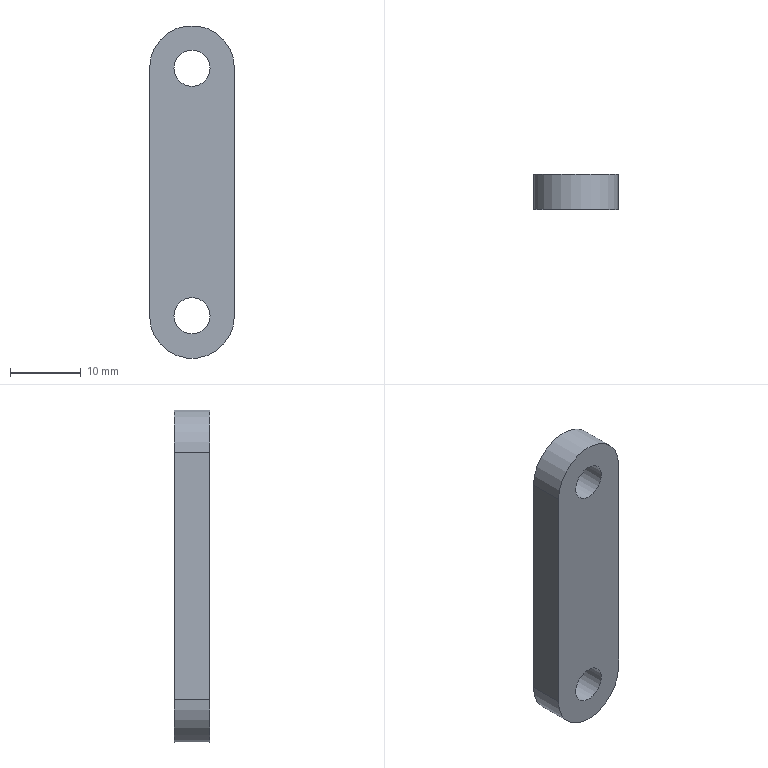Component | NX | SHORT_LINK | 1 solid | 8 faces | box 12 x 5 x 47 mm | volume 2461 mm3 | plane 4 | cylinder 4 | commonest cylinder face diameters 12 x2 5.1 x2
STEP:
#1=CARTESIAN_POINT('',(0.,0.,0.));
#2=DIRECTION('',(0.,0.,1.));
#3=DIRECTION('',(1.,0.,0.));
#4=AXIS2_PLACEMENT_3D('',#1,#2,#3);
#5=CARTESIAN_POINT('',(-34.,3.5,67.45));
#6=VERTEX_POINT('',#5);
#7=CARTESIAN_POINT('',(-34.,3.5,102.45));
#8=VERTEX_POINT('',#7);
#9=CARTESIAN_POINT('',(-34.,3.5,67.45));
#10=DIRECTION('',(-0.,0.,1.));
#11=VECTOR('',#10,1.);
#12=LINE('',#9,#11);
#13=CARTESIAN_POINT('',(-34.,-1.5,67.45));
#14=DIRECTION('',(-1.,0.,-0.));
#15=DIRECTION('',(0.,0.,-1.));
#16=AXIS2_PLACEMENT_3D('',#13,#14,#15);
#17=PLANE('',#16);
#18=CARTESIAN_POINT('',(0.,-5.));
#19=DIRECTION('',(-1.,0.));
#20=VECTOR('',#19,1.);
#21=LINE('',#18,#20);
#22=(GEOMETRIC_REPRESENTATION_CONTEXT(2)PARAMETRIC_REPRESENTATION_CONTEXT()REPRESENTATION_CONTEXT('',''));
#23=DEFINITIONAL_REPRESENTATION('',(#21),#22);
#24=PCURVE('',#17,#23);
#25=CARTESIAN_POINT('',(-40.,3.5,102.45));
#26=DIRECTION('',(0.,-1.,0.));
#27=DIRECTION('',(1.,0.,0.));
#28=AXIS2_PLACEMENT_3D('',#25,#26,#27);
#29=PLANE('',#28);
#30=CARTESIAN_POINT('',(6.,-35.));
#31=DIRECTION('',(-0.,1.));
#32=VECTOR('',#31,1.);
#33=LINE('',#30,#32);
#34=(GEOMETRIC_REPRESENTATION_CONTEXT(2)PARAMETRIC_REPRESENTATION_CONTEXT()REPRESENTATION_CONTEXT('',''));
#35=DEFINITIONAL_REPRESENTATION('',(#33),#34);
#36=PCURVE('',#29,#35);
#37=SURFACE_CURVE('',#12,(#24,#36),.PCURVE_S1.);
#38=EDGE_CURVE('',#6,#8,#37,.T.);
#39=ORIENTED_EDGE('',*,*,#38,.T.);
#40=CARTESIAN_POINT('',(-34.,-1.5,102.45));
#41=VERTEX_POINT('',#40);
#42=CARTESIAN_POINT('',(-34.,-1.5,102.45));
#43=DIRECTION('',(0.,1.,0.));
#44=VECTOR('',#43,1.);
#45=LINE('',#42,#44);
#46=CARTESIAN_POINT('',(-35.,0.));
#47=DIRECTION('',(0.,-1.));
#48=VECTOR('',#47,1.);
#49=LINE('',#46,#48);
#50=(GEOMETRIC_REPRESENTATION_CONTEXT(2)PARAMETRIC_REPRESENTATION_CONTEXT()REPRESENTATION_CONTEXT('',''));
#51=DEFINITIONAL_REPRESENTATION('',(#49),#50);
#52=PCURVE('',#17,#51);
#53=CARTESIAN_POINT('',(-40.,-1.5,102.45));
#54=DIRECTION('',(0.,1.,0.));
#55=DIRECTION('',(-1.,0.,0.));
#56=AXIS2_PLACEMENT_3D('',#53,#54,#55);
#57=CYLINDRICAL_SURFACE('',#56,6.);
#58=CARTESIAN_POINT('',(3.142,0.));
#59=DIRECTION('',(0.,1.));
#60=VECTOR('',#59,1.);
#61=LINE('',#58,#60);
#62=(GEOMETRIC_REPRESENTATION_CONTEXT(2)PARAMETRIC_REPRESENTATION_CONTEXT()REPRESENTATION_CONTEXT('',''));
#63=DEFINITIONAL_REPRESENTATION('',(#61),#62);
#64=PCURVE('',#57,#63);
#65=SURFACE_CURVE('',#45,(#52,#64),.PCURVE_S1.);
#66=EDGE_CURVE('',#41,#8,#65,.T.);
#67=ORIENTED_EDGE('',*,*,#66,.F.);
#68=CARTESIAN_POINT('',(-34.,-1.5,67.45));
#69=VERTEX_POINT('',#68);
#70=CARTESIAN_POINT('',(-34.,-1.5,67.45));
#71=DIRECTION('',(-0.,0.,1.));
#72=VECTOR('',#71,1.);
#73=LINE('',#70,#72);
#74=CARTESIAN_POINT('',(0.,0.));
#75=DIRECTION('',(-1.,0.));
#76=VECTOR('',#75,1.);
#77=LINE('',#74,#76);
#78=(GEOMETRIC_REPRESENTATION_CONTEXT(2)PARAMETRIC_REPRESENTATION_CONTEXT()REPRESENTATION_CONTEXT('',''));
#79=DEFINITIONAL_REPRESENTATION('',(#77),#78);
#80=PCURVE('',#17,#79);
#81=CARTESIAN_POINT('',(-40.,-1.5,102.45));
#82=DIRECTION('',(0.,-1.,0.));
#83=DIRECTION('',(1.,0.,0.));
#84=AXIS2_PLACEMENT_3D('',#81,#82,#83);
#85=PLANE('',#84);
#86=CARTESIAN_POINT('',(6.,-35.));
#87=DIRECTION('',(-0.,1.));
#88=VECTOR('',#87,1.);
#89=LINE('',#86,#88);
#90=(GEOMETRIC_REPRESENTATION_CONTEXT(2)PARAMETRIC_REPRESENTATION_CONTEXT()REPRESENTATION_CONTEXT('',''));
#91=DEFINITIONAL_REPRESENTATION('',(#89),#90);
#92=PCURVE('',#85,#91);
#93=SURFACE_CURVE('',#73,(#80,#92),.PCURVE_S1.);
#94=EDGE_CURVE('',#69,#41,#93,.T.);
#95=ORIENTED_EDGE('',*,*,#94,.F.);
#96=CARTESIAN_POINT('',(-34.,-1.5,67.45));
#97=DIRECTION('',(0.,1.,0.));
#98=VECTOR('',#97,1.);
#99=LINE('',#96,#98);
#100=CARTESIAN_POINT('',(0.,0.));
#101=DIRECTION('',(0.,-1.));
#102=VECTOR('',#101,1.);
#103=LINE('',#100,#102);
#104=(GEOMETRIC_REPRESENTATION_CONTEXT(2)PARAMETRIC_REPRESENTATION_CONTEXT()REPRESENTATION_CONTEXT('',''));
#105=DEFINITIONAL_REPRESENTATION('',(#103),#104);
#106=PCURVE('',#17,#105);
#107=CARTESIAN_POINT('',(-40.,-1.5,67.45));
#108=DIRECTION('',(0.,1.,0.));
#109=DIRECTION('',(-1.,0.,0.));
#110=AXIS2_PLACEMENT_3D('',#107,#108,#109);
#111=CYLINDRICAL_SURFACE('',#110,6.);
#112=CARTESIAN_POINT('',(3.142,0.));
#113=DIRECTION('',(0.,1.));
#114=VECTOR('',#113,1.);
#115=LINE('',#112,#114);
#116=(GEOMETRIC_REPRESENTATION_CONTEXT(2)PARAMETRIC_REPRESENTATION_CONTEXT()REPRESENTATION_CONTEXT('',''));
#117=DEFINITIONAL_REPRESENTATION('',(#115),#116);
#118=PCURVE('',#111,#117);
#119=SURFACE_CURVE('',#99,(#106,#118),.PCURVE_S1.);
#120=EDGE_CURVE('',#69,#6,#119,.T.);
#121=ORIENTED_EDGE('',*,*,#120,.T.);
#122=EDGE_LOOP('',(#39,#67,#95,#121));
#123=FACE_BOUND('',#122,.T.);
#124=ADVANCED_FACE('',(#123),#17,.F.);
#125=CARTESIAN_POINT('',(-46.,3.5,102.45));
#126=VERTEX_POINT('',#125);
#127=CARTESIAN_POINT('',(-40.,3.5,102.45));
#128=DIRECTION('',(0.,-1.,0.));
#129=DIRECTION('',(1.,0.,0.));
#130=AXIS2_PLACEMENT_3D('',#127,#128,#129);
#131=CIRCLE('',#130,6.);
#132=CARTESIAN_POINT('',(3.142,5.));
#133=DIRECTION('',(-1.,0.));
#134=VECTOR('',#133,1.);
#135=LINE('',#132,#134);
#136=(GEOMETRIC_REPRESENTATION_CONTEXT(2)PARAMETRIC_REPRESENTATION_CONTEXT()REPRESENTATION_CONTEXT('',''));
#137=DEFINITIONAL_REPRESENTATION('',(#135),#136);
#138=PCURVE('',#57,#137);
#139=CARTESIAN_POINT('',(0.,0.));
#140=DIRECTION('',(1.,0.));
#141=AXIS2_PLACEMENT_2D('',#139,#140);
#142=CIRCLE('',#141,6.);
#143=(GEOMETRIC_REPRESENTATION_CONTEXT(2)PARAMETRIC_REPRESENTATION_CONTEXT()REPRESENTATION_CONTEXT('',''));
#144=DEFINITIONAL_REPRESENTATION('',(#142),#143);
#145=PCURVE('',#29,#144);
#146=SURFACE_CURVE('',#131,(#138,#145),.PCURVE_S1.);
#147=EDGE_CURVE('',#8,#126,#146,.T.);
#148=ORIENTED_EDGE('',*,*,#147,.T.);
#149=CARTESIAN_POINT('',(-46.,-1.5,102.45));
#150=VERTEX_POINT('',#149);
#151=CARTESIAN_POINT('',(-46.,-1.5,102.45));
#152=DIRECTION('',(0.,1.,0.));
#153=VECTOR('',#152,1.);
#154=LINE('',#151,#153);
#155=CARTESIAN_POINT('',(0.,0.));
#156=DIRECTION('',(0.,1.));
#157=VECTOR('',#156,1.);
#158=LINE('',#155,#157);
#159=(GEOMETRIC_REPRESENTATION_CONTEXT(2)PARAMETRIC_REPRESENTATION_CONTEXT()REPRESENTATION_CONTEXT('',''));
#160=DEFINITIONAL_REPRESENTATION('',(#158),#159);
#161=PCURVE('',#57,#160);
#162=CARTESIAN_POINT('',(-46.,-1.5,102.45));
#163=DIRECTION('',(1.,0.,0.));
#164=DIRECTION('',(-0.,0.,1.));
#165=AXIS2_PLACEMENT_3D('',#162,#163,#164);
#166=PLANE('',#165);
#167=CARTESIAN_POINT('',(0.,0.));
#168=DIRECTION('',(0.,-1.));
#169=VECTOR('',#168,1.);
#170=LINE('',#167,#169);
#171=(GEOMETRIC_REPRESENTATION_CONTEXT(2)PARAMETRIC_REPRESENTATION_CONTEXT()REPRESENTATION_CONTEXT('',''));
#172=DEFINITIONAL_REPRESENTATION('',(#170),#171);
#173=PCURVE('',#166,#172);
#174=SURFACE_CURVE('',#154,(#161,#173),.PCURVE_S1.);
#175=EDGE_CURVE('',#150,#126,#174,.T.);
#176=ORIENTED_EDGE('',*,*,#175,.F.);
#177=CARTESIAN_POINT('',(-40.,-1.5,102.45));
#178=DIRECTION('',(0.,-1.,0.));
#179=DIRECTION('',(1.,0.,0.));
#180=AXIS2_PLACEMENT_3D('',#177,#178,#179);
#181=CIRCLE('',#180,6.);
#182=CARTESIAN_POINT('',(3.142,0.));
#183=DIRECTION('',(-1.,0.));
#184=VECTOR('',#183,1.);
#185=LINE('',#182,#184);
#186=(GEOMETRIC_REPRESENTATION_CONTEXT(2)PARAMETRIC_REPRESENTATION_CONTEXT()REPRESENTATION_CONTEXT('',''));
#187=DEFINITIONAL_REPRESENTATION('',(#185),#186);
#188=PCURVE('',#57,#187);
#189=CARTESIAN_POINT('',(0.,0.));
#190=DIRECTION('',(1.,0.));
#191=AXIS2_PLACEMENT_2D('',#189,#190);
#192=CIRCLE('',#191,6.);
#193=(GEOMETRIC_REPRESENTATION_CONTEXT(2)PARAMETRIC_REPRESENTATION_CONTEXT()REPRESENTATION_CONTEXT('',''));
#194=DEFINITIONAL_REPRESENTATION('',(#192),#193);
#195=PCURVE('',#85,#194);
#196=SURFACE_CURVE('',#181,(#188,#195),.PCURVE_S1.);
#197=EDGE_CURVE('',#41,#150,#196,.T.);
#198=ORIENTED_EDGE('',*,*,#197,.F.);
#199=ORIENTED_EDGE('',*,*,#66,.T.);
#200=EDGE_LOOP('',(#148,#176,#198,#199));
#201=FACE_BOUND('',#200,.T.);
#202=ADVANCED_FACE('',(#201),#57,.T.);
#203=CARTESIAN_POINT('',(-46.,3.5,67.45));
#204=VERTEX_POINT('',#203);
#205=CARTESIAN_POINT('',(-46.,3.5,102.45));
#206=DIRECTION('',(0.,0.,-1.));
#207=VECTOR('',#206,1.);
#208=LINE('',#205,#207);
#209=CARTESIAN_POINT('',(0.,-5.));
#210=DIRECTION('',(-1.,0.));
#211=VECTOR('',#210,1.);
#212=LINE('',#209,#211);
#213=(GEOMETRIC_REPRESENTATION_CONTEXT(2)PARAMETRIC_REPRESENTATION_CONTEXT()REPRESENTATION_CONTEXT('',''));
#214=DEFINITIONAL_REPRESENTATION('',(#212),#213);
#215=PCURVE('',#166,#214);
#216=CARTESIAN_POINT('',(-6.,0.));
#217=DIRECTION('',(0.,-1.));
#218=VECTOR('',#217,1.);
#219=LINE('',#216,#218);
#220=(GEOMETRIC_REPRESENTATION_CONTEXT(2)PARAMETRIC_REPRESENTATION_CONTEXT()REPRESENTATION_CONTEXT('',''));
#221=DEFINITIONAL_REPRESENTATION('',(#219),#220);
#222=PCURVE('',#29,#221);
#223=SURFACE_CURVE('',#208,(#215,#222),.PCURVE_S1.);
#224=EDGE_CURVE('',#126,#204,#223,.T.);
#225=ORIENTED_EDGE('',*,*,#224,.T.);
#226=CARTESIAN_POINT('',(-46.,-1.5,67.45));
#227=VERTEX_POINT('',#226);
#228=CARTESIAN_POINT('',(-46.,-1.5,67.45));
#229=DIRECTION('',(0.,1.,0.));
#230=VECTOR('',#229,1.);
#231=LINE('',#228,#230);
#232=CARTESIAN_POINT('',(-35.,0.));
#233=DIRECTION('',(0.,-1.));
#234=VECTOR('',#233,1.);
#235=LINE('',#232,#234);
#236=(GEOMETRIC_REPRESENTATION_CONTEXT(2)PARAMETRIC_REPRESENTATION_CONTEXT()REPRESENTATION_CONTEXT('',''));
#237=DEFINITIONAL_REPRESENTATION('',(#235),#236);
#238=PCURVE('',#166,#237);
#239=CARTESIAN_POINT('',(6.283,0.));
#240=DIRECTION('',(0.,1.));
#241=VECTOR('',#240,1.);
#242=LINE('',#239,#241);
#243=(GEOMETRIC_REPRESENTATION_CONTEXT(2)PARAMETRIC_REPRESENTATION_CONTEXT()REPRESENTATION_CONTEXT('',''));
#244=DEFINITIONAL_REPRESENTATION('',(#242),#243);
#245=PCURVE('',#111,#244);
#246=SURFACE_CURVE('',#231,(#238,#245),.PCURVE_S1.);
#247=EDGE_CURVE('',#227,#204,#246,.T.);
#248=ORIENTED_EDGE('',*,*,#247,.F.);
#249=CARTESIAN_POINT('',(-46.,-1.5,102.45));
#250=DIRECTION('',(0.,0.,-1.));
#251=VECTOR('',#250,1.);
#252=LINE('',#249,#251);
#253=CARTESIAN_POINT('',(0.,0.));
#254=DIRECTION('',(-1.,0.));
#255=VECTOR('',#254,1.);
#256=LINE('',#253,#255);
#257=(GEOMETRIC_REPRESENTATION_CONTEXT(2)PARAMETRIC_REPRESENTATION_CONTEXT()REPRESENTATION_CONTEXT('',''));
#258=DEFINITIONAL_REPRESENTATION('',(#256),#257);
#259=PCURVE('',#166,#258);
#260=CARTESIAN_POINT('',(-6.,0.));
#261=DIRECTION('',(0.,-1.));
#262=VECTOR('',#261,1.);
#263=LINE('',#260,#262);
#264=(GEOMETRIC_REPRESENTATION_CONTEXT(2)PARAMETRIC_REPRESENTATION_CONTEXT()REPRESENTATION_CONTEXT('',''));
#265=DEFINITIONAL_REPRESENTATION('',(#263),#264);
#266=PCURVE('',#85,#265);
#267=SURFACE_CURVE('',#252,(#259,#266),.PCURVE_S1.);
#268=EDGE_CURVE('',#150,#227,#267,.T.);
#269=ORIENTED_EDGE('',*,*,#268,.F.);
#270=ORIENTED_EDGE('',*,*,#175,.T.);
#271=EDGE_LOOP('',(#225,#248,#269,#270));
#272=FACE_BOUND('',#271,.T.);
#273=ADVANCED_FACE('',(#272),#166,.F.);
#274=CARTESIAN_POINT('',(-37.45,-1.5,102.45));
#275=VERTEX_POINT('',#274);
#276=CARTESIAN_POINT('',(-40.,-1.5,102.45));
#277=DIRECTION('',(0.,1.,0.));
#278=DIRECTION('',(1.,0.,0.));
#279=AXIS2_PLACEMENT_3D('',#276,#277,#278);
#280=CIRCLE('',#279,2.55);
#281=CARTESIAN_POINT('',(-40.,-1.5,102.45));
#282=DIRECTION('',(0.,1.,0.));
#283=DIRECTION('',(-1.,0.,0.));
#284=AXIS2_PLACEMENT_3D('',#281,#282,#283);
#285=CYLINDRICAL_SURFACE('',#284,2.55);
#286=CARTESIAN_POINT('',(3.142,0.));
#287=DIRECTION('',(1.,0.));
#288=VECTOR('',#287,1.);
#289=LINE('',#286,#288);
#290=(GEOMETRIC_REPRESENTATION_CONTEXT(2)PARAMETRIC_REPRESENTATION_CONTEXT()REPRESENTATION_CONTEXT('',''));
#291=DEFINITIONAL_REPRESENTATION('',(#289),#290);
#292=PCURVE('',#285,#291);
#293=CARTESIAN_POINT('',(2.55,0.));
#294=CARTESIAN_POINT('',(2.55,-4.417));
#295=CARTESIAN_POINT('',(-1.275,-2.208));
#296=CARTESIAN_POINT('',(-5.1,-0.));
#297=CARTESIAN_POINT('',(-1.275,2.208));
#298=CARTESIAN_POINT('',(2.55,4.417));
#299=CARTESIAN_POINT('',(2.55,0.));
#300=(BOUNDED_CURVE()B_SPLINE_CURVE(2,(#293,#294,#295,#296,#297,#298,#299),.UNSPECIFIED.,.T.,.F.)B_SPLINE_CURVE_WITH_KNOTS((1,2,2,2,2,1),(-2.094,0.,2.094,4.189,6.283,8.378),.UNSPECIFIED.)CURVE()GEOMETRIC_REPRESENTATION_ITEM()RATIONAL_B_SPLINE_CURVE((1.,0.5,1.,0.5,1.,0.5,1.))REPRESENTATION_ITEM(''));
#301=(GEOMETRIC_REPRESENTATION_CONTEXT(2)PARAMETRIC_REPRESENTATION_CONTEXT()REPRESENTATION_CONTEXT('',''));
#302=DEFINITIONAL_REPRESENTATION('',(#300),#301);
#303=PCURVE('',#85,#302);
#304=SURFACE_CURVE('',#280,(#292,#303),.PCURVE_S1.);
#305=EDGE_CURVE('',#275,#275,#304,.T.);
#306=ORIENTED_EDGE('',*,*,#305,.T.);
#307=CARTESIAN_POINT('',(-37.45,3.5,102.45));
#308=VERTEX_POINT('',#307);
#309=CARTESIAN_POINT('',(-37.45,-1.5,102.45));
#310=CARTESIAN_POINT('',(-37.45,3.5,102.45));
#311=B_SPLINE_CURVE_WITH_KNOTS('',1,(#309,#310),.UNSPECIFIED.,.F.,.F.,(2,2),(0.,5.),.PIECEWISE_BEZIER_KNOTS.);
#312=CARTESIAN_POINT('',(9.425,0.));
#313=DIRECTION('',(0.,1.));
#314=VECTOR('',#313,1.);
#315=LINE('',#312,#314);
#316=(GEOMETRIC_REPRESENTATION_CONTEXT(2)PARAMETRIC_REPRESENTATION_CONTEXT()REPRESENTATION_CONTEXT('',''));
#317=DEFINITIONAL_REPRESENTATION('',(#315),#316);
#318=PCURVE('',#285,#317);
#319=CARTESIAN_POINT('',(3.142,0.));
#320=DIRECTION('',(0.,1.));
#321=VECTOR('',#320,1.);
#322=LINE('',#319,#321);
#323=(GEOMETRIC_REPRESENTATION_CONTEXT(2)PARAMETRIC_REPRESENTATION_CONTEXT()REPRESENTATION_CONTEXT('',''));
#324=DEFINITIONAL_REPRESENTATION('',(#322),#323);
#325=PCURVE('',#285,#324);
#326=SEAM_CURVE('',#311,(#318,#325),.PCURVE_S1.);
#327=EDGE_CURVE('',#275,#308,#326,.T.);
#328=ORIENTED_EDGE('',*,*,#327,.T.);
#329=CARTESIAN_POINT('',(-40.,3.5,102.45));
#330=DIRECTION('',(0.,1.,0.));
#331=DIRECTION('',(1.,0.,0.));
#332=AXIS2_PLACEMENT_3D('',#329,#330,#331);
#333=CIRCLE('',#332,2.55);
#334=CARTESIAN_POINT('',(3.142,5.));
#335=DIRECTION('',(1.,0.));
#336=VECTOR('',#335,1.);
#337=LINE('',#334,#336);
#338=(GEOMETRIC_REPRESENTATION_CONTEXT(2)PARAMETRIC_REPRESENTATION_CONTEXT()REPRESENTATION_CONTEXT('',''));
#339=DEFINITIONAL_REPRESENTATION('',(#337),#338);
#340=PCURVE('',#285,#339);
#341=CARTESIAN_POINT('',(2.55,0.));
#342=CARTESIAN_POINT('',(2.55,-4.417));
#343=CARTESIAN_POINT('',(-1.275,-2.208));
#344=CARTESIAN_POINT('',(-5.1,-0.));
#345=CARTESIAN_POINT('',(-1.275,2.208));
#346=CARTESIAN_POINT('',(2.55,4.417));
#347=CARTESIAN_POINT('',(2.55,0.));
#348=(BOUNDED_CURVE()B_SPLINE_CURVE(2,(#341,#342,#343,#344,#345,#346,#347),.UNSPECIFIED.,.T.,.F.)B_SPLINE_CURVE_WITH_KNOTS((1,2,2,2,2,1),(-2.094,0.,2.094,4.189,6.283,8.378),.UNSPECIFIED.)CURVE()GEOMETRIC_REPRESENTATION_ITEM()RATIONAL_B_SPLINE_CURVE((1.,0.5,1.,0.5,1.,0.5,1.))REPRESENTATION_ITEM(''));
#349=(GEOMETRIC_REPRESENTATION_CONTEXT(2)PARAMETRIC_REPRESENTATION_CONTEXT()REPRESENTATION_CONTEXT('',''));
#350=DEFINITIONAL_REPRESENTATION('',(#348),#349);
#351=PCURVE('',#29,#350);
#352=SURFACE_CURVE('',#333,(#340,#351),.PCURVE_S1.);
#353=EDGE_CURVE('',#308,#308,#352,.T.);
#354=ORIENTED_EDGE('',*,*,#353,.F.);
#355=ORIENTED_EDGE('',*,*,#327,.F.);
#356=EDGE_LOOP('',(#306,#328,#354,#355));
#357=FACE_BOUND('',#356,.F.);
#358=ADVANCED_FACE('',(#357),#285,.F.);
#359=CARTESIAN_POINT('',(-40.,3.5,67.45));
#360=DIRECTION('',(0.,-1.,0.));
#361=DIRECTION('',(1.,0.,0.));
#362=AXIS2_PLACEMENT_3D('',#359,#360,#361);
#363=CIRCLE('',#362,6.);
#364=CARTESIAN_POINT('',(9.425,5.));
#365=DIRECTION('',(-1.,0.));
#366=VECTOR('',#365,1.);
#367=LINE('',#364,#366);
#368=(GEOMETRIC_REPRESENTATION_CONTEXT(2)PARAMETRIC_REPRESENTATION_CONTEXT()REPRESENTATION_CONTEXT('',''));
#369=DEFINITIONAL_REPRESENTATION('',(#367),#368);
#370=PCURVE('',#111,#369);
#371=CARTESIAN_POINT('',(0.,-35.));
#372=DIRECTION('',(1.,0.));
#373=AXIS2_PLACEMENT_2D('',#371,#372);
#374=CIRCLE('',#373,6.);
#375=(GEOMETRIC_REPRESENTATION_CONTEXT(2)PARAMETRIC_REPRESENTATION_CONTEXT()REPRESENTATION_CONTEXT('',''));
#376=DEFINITIONAL_REPRESENTATION('',(#374),#375);
#377=PCURVE('',#29,#376);
#378=SURFACE_CURVE('',#363,(#370,#377),.PCURVE_S1.);
#379=EDGE_CURVE('',#204,#6,#378,.T.);
#380=ORIENTED_EDGE('',*,*,#379,.T.);
#381=ORIENTED_EDGE('',*,*,#120,.F.);
#382=CARTESIAN_POINT('',(-40.,-1.5,67.45));
#383=DIRECTION('',(0.,-1.,0.));
#384=DIRECTION('',(1.,0.,0.));
#385=AXIS2_PLACEMENT_3D('',#382,#383,#384);
#386=CIRCLE('',#385,6.);
#387=CARTESIAN_POINT('',(9.425,0.));
#388=DIRECTION('',(-1.,0.));
#389=VECTOR('',#388,1.);
#390=LINE('',#387,#389);
#391=(GEOMETRIC_REPRESENTATION_CONTEXT(2)PARAMETRIC_REPRESENTATION_CONTEXT()REPRESENTATION_CONTEXT('',''));
#392=DEFINITIONAL_REPRESENTATION('',(#390),#391);
#393=PCURVE('',#111,#392);
#394=CARTESIAN_POINT('',(0.,-35.));
#395=DIRECTION('',(1.,0.));
#396=AXIS2_PLACEMENT_2D('',#394,#395);
#397=CIRCLE('',#396,6.);
#398=(GEOMETRIC_REPRESENTATION_CONTEXT(2)PARAMETRIC_REPRESENTATION_CONTEXT()REPRESENTATION_CONTEXT('',''));
#399=DEFINITIONAL_REPRESENTATION('',(#397),#398);
#400=PCURVE('',#85,#399);
#401=SURFACE_CURVE('',#386,(#393,#400),.PCURVE_S1.);
#402=EDGE_CURVE('',#227,#69,#401,.T.);
#403=ORIENTED_EDGE('',*,*,#402,.F.);
#404=ORIENTED_EDGE('',*,*,#247,.T.);
#405=EDGE_LOOP('',(#380,#381,#403,#404));
#406=FACE_BOUND('',#405,.T.);
#407=ADVANCED_FACE('',(#406),#111,.T.);
#408=CARTESIAN_POINT('',(-37.45,-1.5,67.45));
#409=VERTEX_POINT('',#408);
#410=CARTESIAN_POINT('',(-40.,-1.5,67.45));
#411=DIRECTION('',(0.,1.,0.));
#412=DIRECTION('',(1.,0.,0.));
#413=AXIS2_PLACEMENT_3D('',#410,#411,#412);
#414=CIRCLE('',#413,2.55);
#415=CARTESIAN_POINT('',(-40.,-1.5,67.45));
#416=DIRECTION('',(0.,1.,0.));
#417=DIRECTION('',(-1.,0.,0.));
#418=AXIS2_PLACEMENT_3D('',#415,#416,#417);
#419=CYLINDRICAL_SURFACE('',#418,2.55);
#420=CARTESIAN_POINT('',(3.142,0.));
#421=DIRECTION('',(1.,0.));
#422=VECTOR('',#421,1.);
#423=LINE('',#420,#422);
#424=(GEOMETRIC_REPRESENTATION_CONTEXT(2)PARAMETRIC_REPRESENTATION_CONTEXT()REPRESENTATION_CONTEXT('',''));
#425=DEFINITIONAL_REPRESENTATION('',(#423),#424);
#426=PCURVE('',#419,#425);
#427=CARTESIAN_POINT('',(2.55,-35.));
#428=CARTESIAN_POINT('',(2.55,-39.417));
#429=CARTESIAN_POINT('',(-1.275,-37.208));
#430=CARTESIAN_POINT('',(-5.1,-35.));
#431=CARTESIAN_POINT('',(-1.275,-32.792));
#432=CARTESIAN_POINT('',(2.55,-30.583));
#433=CARTESIAN_POINT('',(2.55,-35.));
#434=(BOUNDED_CURVE()B_SPLINE_CURVE(2,(#427,#428,#429,#430,#431,#432,#433),.UNSPECIFIED.,.T.,.F.)B_SPLINE_CURVE_WITH_KNOTS((1,2,2,2,2,1),(-2.094,0.,2.094,4.189,6.283,8.378),.UNSPECIFIED.)CURVE()GEOMETRIC_REPRESENTATION_ITEM()RATIONAL_B_SPLINE_CURVE((1.,0.5,1.,0.5,1.,0.5,1.))REPRESENTATION_ITEM(''));
#435=(GEOMETRIC_REPRESENTATION_CONTEXT(2)PARAMETRIC_REPRESENTATION_CONTEXT()REPRESENTATION_CONTEXT('',''));
#436=DEFINITIONAL_REPRESENTATION('',(#434),#435);
#437=PCURVE('',#85,#436);
#438=SURFACE_CURVE('',#414,(#426,#437),.PCURVE_S1.);
#439=EDGE_CURVE('',#409,#409,#438,.T.);
#440=ORIENTED_EDGE('',*,*,#439,.T.);
#441=CARTESIAN_POINT('',(-37.45,3.5,67.45));
#442=VERTEX_POINT('',#441);
#443=CARTESIAN_POINT('',(-37.45,-1.5,67.45));
#444=CARTESIAN_POINT('',(-37.45,3.5,67.45));
#445=B_SPLINE_CURVE_WITH_KNOTS('',1,(#443,#444),.UNSPECIFIED.,.F.,.F.,(2,2),(0.,5.),.PIECEWISE_BEZIER_KNOTS.);
#446=CARTESIAN_POINT('',(9.425,0.));
#447=DIRECTION('',(0.,1.));
#448=VECTOR('',#447,1.);
#449=LINE('',#446,#448);
#450=(GEOMETRIC_REPRESENTATION_CONTEXT(2)PARAMETRIC_REPRESENTATION_CONTEXT()REPRESENTATION_CONTEXT('',''));
#451=DEFINITIONAL_REPRESENTATION('',(#449),#450);
#452=PCURVE('',#419,#451);
#453=CARTESIAN_POINT('',(3.142,0.));
#454=DIRECTION('',(0.,1.));
#455=VECTOR('',#454,1.);
#456=LINE('',#453,#455);
#457=(GEOMETRIC_REPRESENTATION_CONTEXT(2)PARAMETRIC_REPRESENTATION_CONTEXT()REPRESENTATION_CONTEXT('',''));
#458=DEFINITIONAL_REPRESENTATION('',(#456),#457);
#459=PCURVE('',#419,#458);
#460=SEAM_CURVE('',#445,(#452,#459),.PCURVE_S1.);
#461=EDGE_CURVE('',#409,#442,#460,.T.);
#462=ORIENTED_EDGE('',*,*,#461,.T.);
#463=CARTESIAN_POINT('',(-40.,3.5,67.45));
#464=DIRECTION('',(0.,1.,0.));
#465=DIRECTION('',(1.,0.,0.));
#466=AXIS2_PLACEMENT_3D('',#463,#464,#465);
#467=CIRCLE('',#466,2.55);
#468=CARTESIAN_POINT('',(3.142,5.));
#469=DIRECTION('',(1.,0.));
#470=VECTOR('',#469,1.);
#471=LINE('',#468,#470);
#472=(GEOMETRIC_REPRESENTATION_CONTEXT(2)PARAMETRIC_REPRESENTATION_CONTEXT()REPRESENTATION_CONTEXT('',''));
#473=DEFINITIONAL_REPRESENTATION('',(#471),#472);
#474=PCURVE('',#419,#473);
#475=CARTESIAN_POINT('',(2.55,-35.));
#476=CARTESIAN_POINT('',(2.55,-39.417));
#477=CARTESIAN_POINT('',(-1.275,-37.208));
#478=CARTESIAN_POINT('',(-5.1,-35.));
#479=CARTESIAN_POINT('',(-1.275,-32.792));
#480=CARTESIAN_POINT('',(2.55,-30.583));
#481=CARTESIAN_POINT('',(2.55,-35.));
#482=(BOUNDED_CURVE()B_SPLINE_CURVE(2,(#475,#476,#477,#478,#479,#480,#481),.UNSPECIFIED.,.T.,.F.)B_SPLINE_CURVE_WITH_KNOTS((1,2,2,2,2,1),(-2.094,0.,2.094,4.189,6.283,8.378),.UNSPECIFIED.)CURVE()GEOMETRIC_REPRESENTATION_ITEM()RATIONAL_B_SPLINE_CURVE((1.,0.5,1.,0.5,1.,0.5,1.))REPRESENTATION_ITEM(''));
#483=(GEOMETRIC_REPRESENTATION_CONTEXT(2)PARAMETRIC_REPRESENTATION_CONTEXT()REPRESENTATION_CONTEXT('',''));
#484=DEFINITIONAL_REPRESENTATION('',(#482),#483);
#485=PCURVE('',#29,#484);
#486=SURFACE_CURVE('',#467,(#474,#485),.PCURVE_S1.);
#487=EDGE_CURVE('',#442,#442,#486,.T.);
#488=ORIENTED_EDGE('',*,*,#487,.F.);
#489=ORIENTED_EDGE('',*,*,#461,.F.);
#490=EDGE_LOOP('',(#440,#462,#488,#489));
#491=FACE_BOUND('',#490,.F.);
#492=ADVANCED_FACE('',(#491),#419,.F.);
#493=ORIENTED_EDGE('',*,*,#94,.T.);
#494=ORIENTED_EDGE('',*,*,#197,.T.);
#495=ORIENTED_EDGE('',*,*,#268,.T.);
#496=ORIENTED_EDGE('',*,*,#402,.T.);
#497=EDGE_LOOP('',(#493,#494,#495,#496));
#498=FACE_BOUND('',#497,.T.);
#499=ORIENTED_EDGE('',*,*,#305,.T.);
#500=EDGE_LOOP('',(#499));
#501=FACE_BOUND('',#500,.T.);
#502=ORIENTED_EDGE('',*,*,#439,.T.);
#503=EDGE_LOOP('',(#502));
#504=FACE_BOUND('',#503,.T.);
#505=ADVANCED_FACE('',(#498,#501,#504),#85,.T.);
#506=ORIENTED_EDGE('',*,*,#38,.F.);
#507=ORIENTED_EDGE('',*,*,#379,.F.);
#508=ORIENTED_EDGE('',*,*,#224,.F.);
#509=ORIENTED_EDGE('',*,*,#147,.F.);
#510=EDGE_LOOP('',(#506,#507,#508,#509));
#511=FACE_BOUND('',#510,.T.);
#512=ORIENTED_EDGE('',*,*,#353,.F.);
#513=EDGE_LOOP('',(#512));
#514=FACE_BOUND('',#513,.T.);
#515=ORIENTED_EDGE('',*,*,#487,.F.);
#516=EDGE_LOOP('',(#515));
#517=FACE_BOUND('',#516,.T.);
#518=ADVANCED_FACE('',(#511,#514,#517),#29,.F.);
#519=CLOSED_SHELL('',(#124,#202,#273,#358,#407,#492,#505,#518));
#520=MANIFOLD_SOLID_BREP('',#519);
#521=(LENGTH_UNIT()NAMED_UNIT(*)SI_UNIT(.MILLI.,.METRE.));
#522=UNCERTAINTY_MEASURE_WITH_UNIT(LENGTH_MEASURE(0.000002),#521,'','');
#523=(NAMED_UNIT(*)PLANE_ANGLE_UNIT()SI_UNIT($,.RADIAN.));
#524=(NAMED_UNIT(*)SI_UNIT($,.STERADIAN.)SOLID_ANGLE_UNIT());
#525=(GEOMETRIC_REPRESENTATION_CONTEXT(3)GLOBAL_UNCERTAINTY_ASSIGNED_CONTEXT((#522))GLOBAL_UNIT_ASSIGNED_CONTEXT((#521,#523,#524))REPRESENTATION_CONTEXT('',''));
#526=ADVANCED_BREP_SHAPE_REPRESENTATION('',(#4,#520),#525);